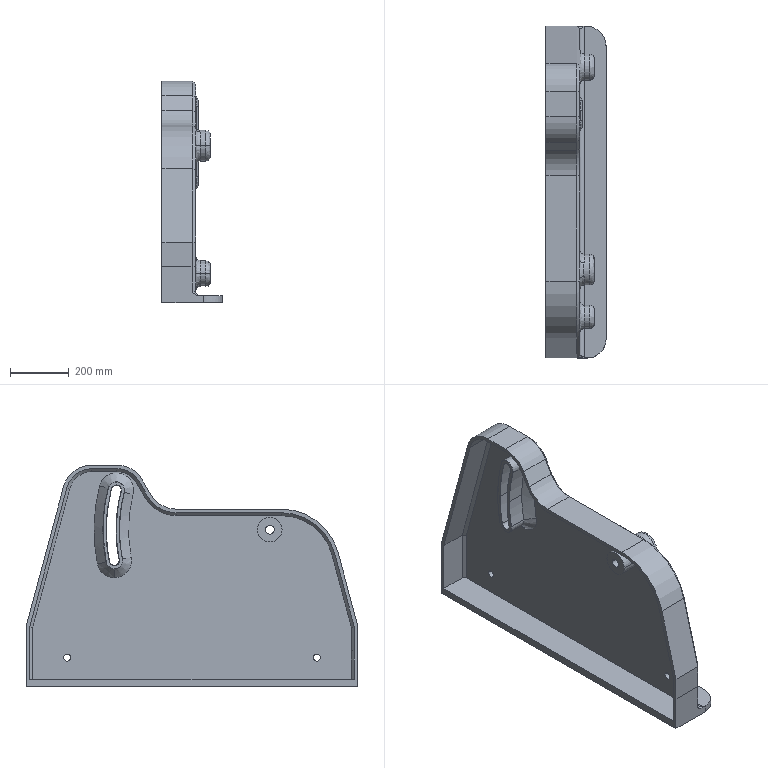Component | SolidWorks | RightBase-1 | 1 solid | 139 faces | volume 21152075 mm3 | cylinder 48 | plane 45 | cone 24 | spline 22 | commonest cylinder face diameters 20 x8 30 x5 24 x4 200 x3 83.378 x2 1023 x2 1137 x2 79.335 x2